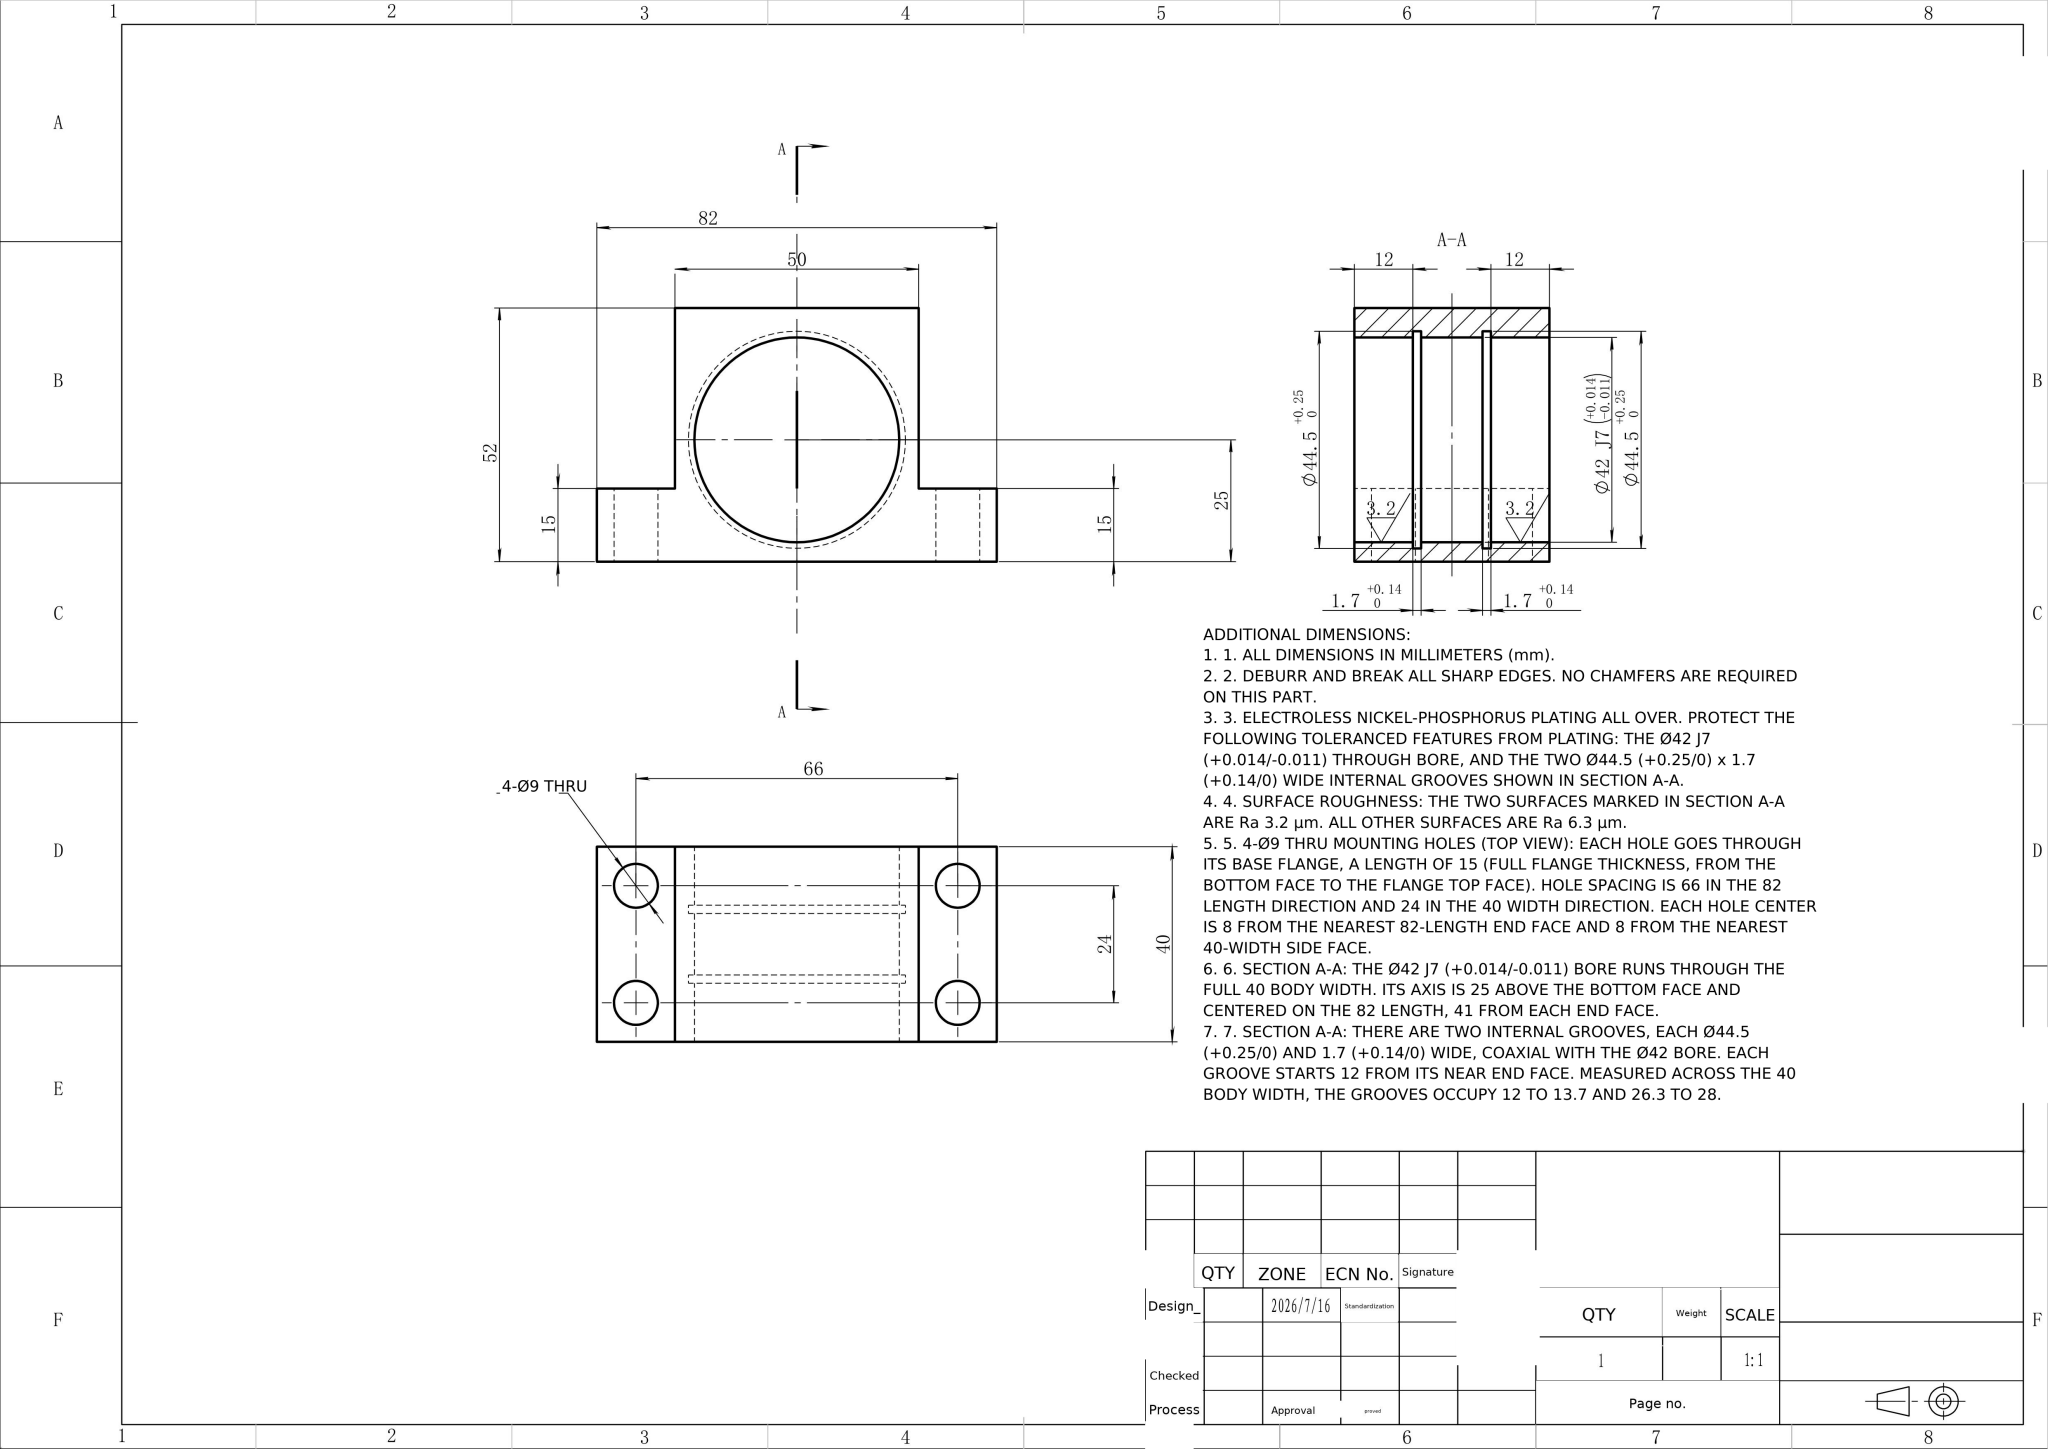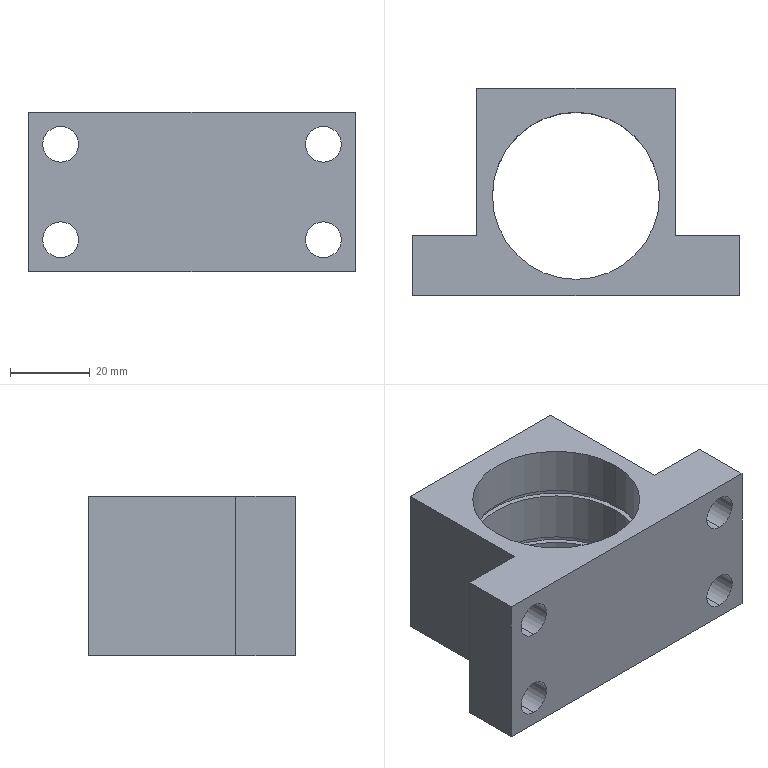Part | NX | mm | 1 solid | 32 faces | box 82 x 52 x 40 mm | volume 63388 mm3 | cylinder 18 | plane 14 | commonest cylinder face diameters 9 x8 42 x6 44.5 x4
STEP:
#1=COLOUR_RGB('',1.,1.,1.);
#2=FILL_AREA_STYLE_COLOUR('',#1);
#3=FILL_AREA_STYLE('',(#2));
#4=SURFACE_STYLE_FILL_AREA(#3);
#5=SURFACE_SIDE_STYLE('',(#4));
#6=SURFACE_STYLE_USAGE(.BOTH.,#5);
#7=PRESENTATION_STYLE_ASSIGNMENT((#6));
#8=CARTESIAN_POINT('',(74.,0.,27.5));
#9=VERTEX_POINT('',#8);
#10=CARTESIAN_POINT('',(74.,0.,36.5));
#11=VERTEX_POINT('',#10);
#12=CARTESIAN_POINT('',(74.,0.,32.));
#13=DIRECTION('',(0.,1.,0.));
#14=DIRECTION('',(0.,0.,-1.));
#15=AXIS2_PLACEMENT_3D('',#12,#13,#14);
#16=CIRCLE('',#15,4.5);
#17=EDGE_CURVE('',#9,#11,#16,.T.);
#18=ORIENTED_EDGE('',*,*,#17,.F.);
#19=CARTESIAN_POINT('',(74.,15.,27.5));
#20=VERTEX_POINT('',#19);
#21=CARTESIAN_POINT('',(74.,-0.001,27.5));
#22=DIRECTION('',(0.,1.,0.));
#23=VECTOR('',#22,1000.);
#24=LINE('',#21,#23);
#25=EDGE_CURVE('',#9,#20,#24,.T.);
#26=ORIENTED_EDGE('',*,*,#25,.T.);
#27=CARTESIAN_POINT('',(74.,15.,36.5));
#28=VERTEX_POINT('',#27);
#29=CARTESIAN_POINT('',(74.,15.,32.));
#30=DIRECTION('',(0.,1.,0.));
#31=DIRECTION('',(0.,0.,1.));
#32=AXIS2_PLACEMENT_3D('',#29,#30,#31);
#33=CIRCLE('',#32,4.5);
#34=EDGE_CURVE('',#20,#28,#33,.T.);
#35=ORIENTED_EDGE('',*,*,#34,.T.);
#36=CARTESIAN_POINT('',(74.,-0.001,36.5));
#37=DIRECTION('',(0.,1.,0.));
#38=VECTOR('',#37,1000.);
#39=LINE('',#36,#38);
#40=EDGE_CURVE('',#11,#28,#39,.T.);
#41=ORIENTED_EDGE('',*,*,#40,.F.);
#42=EDGE_LOOP('',(#18,#26,#35,#41));
#43=FACE_OUTER_BOUND('',#42,.T.);
#44=CARTESIAN_POINT('',(74.,-0.001,32.));
#45=DIRECTION('',(0.,1.,0.));
#46=DIRECTION('',(0.,0.,1.));
#47=AXIS2_PLACEMENT_3D('',#44,#45,#46);
#48=CYLINDRICAL_SURFACE('',#47,4.5);
#49=ADVANCED_FACE('',(#43),#48,.F.);
#50=CARTESIAN_POINT('',(74.,0.,3.5));
#51=VERTEX_POINT('',#50);
#52=CARTESIAN_POINT('',(74.,0.,12.5));
#53=VERTEX_POINT('',#52);
#54=CARTESIAN_POINT('',(74.,0.,8.));
#55=DIRECTION('',(0.,1.,0.));
#56=DIRECTION('',(0.,0.,-1.));
#57=AXIS2_PLACEMENT_3D('',#54,#55,#56);
#58=CIRCLE('',#57,4.5);
#59=EDGE_CURVE('',#51,#53,#58,.T.);
#60=ORIENTED_EDGE('',*,*,#59,.F.);
#61=CARTESIAN_POINT('',(74.,15.,3.5));
#62=VERTEX_POINT('',#61);
#63=CARTESIAN_POINT('',(74.,-0.001,3.5));
#64=DIRECTION('',(0.,1.,0.));
#65=VECTOR('',#64,1000.);
#66=LINE('',#63,#65);
#67=EDGE_CURVE('',#51,#62,#66,.T.);
#68=ORIENTED_EDGE('',*,*,#67,.T.);
#69=CARTESIAN_POINT('',(74.,15.,12.5));
#70=VERTEX_POINT('',#69);
#71=CARTESIAN_POINT('',(74.,15.,8.));
#72=DIRECTION('',(0.,1.,0.));
#73=DIRECTION('',(0.,0.,1.));
#74=AXIS2_PLACEMENT_3D('',#71,#72,#73);
#75=CIRCLE('',#74,4.5);
#76=EDGE_CURVE('',#62,#70,#75,.T.);
#77=ORIENTED_EDGE('',*,*,#76,.T.);
#78=CARTESIAN_POINT('',(74.,-0.001,12.5));
#79=DIRECTION('',(0.,1.,0.));
#80=VECTOR('',#79,1000.);
#81=LINE('',#78,#80);
#82=EDGE_CURVE('',#53,#70,#81,.T.);
#83=ORIENTED_EDGE('',*,*,#82,.F.);
#84=EDGE_LOOP('',(#60,#68,#77,#83));
#85=FACE_OUTER_BOUND('',#84,.T.);
#86=CARTESIAN_POINT('',(74.,-0.001,8.));
#87=DIRECTION('',(0.,1.,0.));
#88=DIRECTION('',(0.,0.,1.));
#89=AXIS2_PLACEMENT_3D('',#86,#87,#88);
#90=CYLINDRICAL_SURFACE('',#89,4.5);
#91=ADVANCED_FACE('',(#85),#90,.F.);
#92=CARTESIAN_POINT('',(8.,0.,27.5));
#93=VERTEX_POINT('',#92);
#94=CARTESIAN_POINT('',(8.,0.,36.5));
#95=VERTEX_POINT('',#94);
#96=CARTESIAN_POINT('',(8.,0.,32.));
#97=DIRECTION('',(0.,1.,0.));
#98=DIRECTION('',(0.,0.,-1.));
#99=AXIS2_PLACEMENT_3D('',#96,#97,#98);
#100=CIRCLE('',#99,4.5);
#101=EDGE_CURVE('',#93,#95,#100,.T.);
#102=ORIENTED_EDGE('',*,*,#101,.F.);
#103=CARTESIAN_POINT('',(8.,15.,27.5));
#104=VERTEX_POINT('',#103);
#105=CARTESIAN_POINT('',(8.,-0.001,27.5));
#106=DIRECTION('',(0.,1.,0.));
#107=VECTOR('',#106,1000.);
#108=LINE('',#105,#107);
#109=EDGE_CURVE('',#93,#104,#108,.T.);
#110=ORIENTED_EDGE('',*,*,#109,.T.);
#111=CARTESIAN_POINT('',(8.,15.,36.5));
#112=VERTEX_POINT('',#111);
#113=CARTESIAN_POINT('',(8.,15.,32.));
#114=DIRECTION('',(0.,1.,0.));
#115=DIRECTION('',(0.,0.,1.));
#116=AXIS2_PLACEMENT_3D('',#113,#114,#115);
#117=CIRCLE('',#116,4.5);
#118=EDGE_CURVE('',#104,#112,#117,.T.);
#119=ORIENTED_EDGE('',*,*,#118,.T.);
#120=CARTESIAN_POINT('',(8.,-0.001,36.5));
#121=DIRECTION('',(0.,1.,0.));
#122=VECTOR('',#121,1000.);
#123=LINE('',#120,#122);
#124=EDGE_CURVE('',#95,#112,#123,.T.);
#125=ORIENTED_EDGE('',*,*,#124,.F.);
#126=EDGE_LOOP('',(#102,#110,#119,#125));
#127=FACE_OUTER_BOUND('',#126,.T.);
#128=CARTESIAN_POINT('',(8.,-0.001,32.));
#129=DIRECTION('',(0.,1.,0.));
#130=DIRECTION('',(0.,0.,1.));
#131=AXIS2_PLACEMENT_3D('',#128,#129,#130);
#132=CYLINDRICAL_SURFACE('',#131,4.5);
#133=ADVANCED_FACE('',(#127),#132,.F.);
#134=CARTESIAN_POINT('',(8.,0.,3.5));
#135=VERTEX_POINT('',#134);
#136=CARTESIAN_POINT('',(8.,0.,12.5));
#137=VERTEX_POINT('',#136);
#138=CARTESIAN_POINT('',(8.,0.,8.));
#139=DIRECTION('',(0.,1.,0.));
#140=DIRECTION('',(0.,0.,-1.));
#141=AXIS2_PLACEMENT_3D('',#138,#139,#140);
#142=CIRCLE('',#141,4.5);
#143=EDGE_CURVE('',#135,#137,#142,.T.);
#144=ORIENTED_EDGE('',*,*,#143,.F.);
#145=CARTESIAN_POINT('',(8.,15.,3.5));
#146=VERTEX_POINT('',#145);
#147=CARTESIAN_POINT('',(8.,-0.001,3.5));
#148=DIRECTION('',(0.,1.,0.));
#149=VECTOR('',#148,1000.);
#150=LINE('',#147,#149);
#151=EDGE_CURVE('',#135,#146,#150,.T.);
#152=ORIENTED_EDGE('',*,*,#151,.T.);
#153=CARTESIAN_POINT('',(8.,15.,12.5));
#154=VERTEX_POINT('',#153);
#155=CARTESIAN_POINT('',(8.,15.,8.));
#156=DIRECTION('',(0.,1.,0.));
#157=DIRECTION('',(0.,0.,1.));
#158=AXIS2_PLACEMENT_3D('',#155,#156,#157);
#159=CIRCLE('',#158,4.5);
#160=EDGE_CURVE('',#146,#154,#159,.T.);
#161=ORIENTED_EDGE('',*,*,#160,.T.);
#162=CARTESIAN_POINT('',(8.,-0.001,12.5));
#163=DIRECTION('',(0.,1.,0.));
#164=VECTOR('',#163,1000.);
#165=LINE('',#162,#164);
#166=EDGE_CURVE('',#137,#154,#165,.T.);
#167=ORIENTED_EDGE('',*,*,#166,.F.);
#168=EDGE_LOOP('',(#144,#152,#161,#167));
#169=FACE_OUTER_BOUND('',#168,.T.);
#170=CARTESIAN_POINT('',(8.,-0.001,8.));
#171=DIRECTION('',(0.,1.,0.));
#172=DIRECTION('',(0.,0.,1.));
#173=AXIS2_PLACEMENT_3D('',#170,#171,#172);
#174=CYLINDRICAL_SURFACE('',#173,4.5);
#175=ADVANCED_FACE('',(#169),#174,.F.);
#176=CARTESIAN_POINT('',(20.,25.,0.));
#177=VERTEX_POINT('',#176);
#178=CARTESIAN_POINT('',(62.,25.,0.));
#179=VERTEX_POINT('',#178);
#180=CARTESIAN_POINT('',(41.,25.,0.));
#181=DIRECTION('',(0.,0.,1.));
#182=DIRECTION('',(1.,0.,0.));
#183=AXIS2_PLACEMENT_3D('',#180,#181,#182);
#184=CIRCLE('',#183,21.);
#185=EDGE_CURVE('',#177,#179,#184,.T.);
#186=ORIENTED_EDGE('',*,*,#185,.F.);
#187=CARTESIAN_POINT('',(20.,25.,12.));
#188=VERTEX_POINT('',#187);
#189=CARTESIAN_POINT('',(20.,25.,0.));
#190=DIRECTION('',(0.,0.,1.));
#191=VECTOR('',#190,1000.);
#192=LINE('',#189,#191);
#193=EDGE_CURVE('',#177,#188,#192,.T.);
#194=ORIENTED_EDGE('',*,*,#193,.T.);
#195=CARTESIAN_POINT('',(62.,25.,12.));
#196=VERTEX_POINT('',#195);
#197=CARTESIAN_POINT('',(41.,25.,12.));
#198=DIRECTION('',(0.,0.,1.));
#199=DIRECTION('',(1.,0.,0.));
#200=AXIS2_PLACEMENT_3D('',#197,#198,#199);
#201=CIRCLE('',#200,21.);
#202=EDGE_CURVE('',#188,#196,#201,.T.);
#203=ORIENTED_EDGE('',*,*,#202,.T.);
#204=CARTESIAN_POINT('',(62.,25.,0.));
#205=DIRECTION('',(0.,0.,1.));
#206=VECTOR('',#205,1000.);
#207=LINE('',#204,#206);
#208=EDGE_CURVE('',#179,#196,#207,.T.);
#209=ORIENTED_EDGE('',*,*,#208,.F.);
#210=EDGE_LOOP('',(#186,#194,#203,#209));
#211=FACE_OUTER_BOUND('',#210,.T.);
#212=CARTESIAN_POINT('',(41.,25.,0.));
#213=DIRECTION('',(0.,0.,1.));
#214=DIRECTION('',(1.,0.,0.));
#215=AXIS2_PLACEMENT_3D('',#212,#213,#214);
#216=CYLINDRICAL_SURFACE('',#215,21.);
#217=ADVANCED_FACE('',(#211),#216,.F.);
#218=CARTESIAN_POINT('',(18.75,25.,12.));
#219=VERTEX_POINT('',#218);
#220=CARTESIAN_POINT('',(63.25,25.,12.));
#221=VERTEX_POINT('',#220);
#222=CARTESIAN_POINT('',(41.,25.,12.));
#223=DIRECTION('',(0.,0.,1.));
#224=DIRECTION('',(1.,0.,0.));
#225=AXIS2_PLACEMENT_3D('',#222,#223,#224);
#226=CIRCLE('',#225,22.25);
#227=EDGE_CURVE('',#219,#221,#226,.T.);
#228=ORIENTED_EDGE('',*,*,#227,.F.);
#229=CARTESIAN_POINT('',(18.75,25.,13.7));
#230=VERTEX_POINT('',#229);
#231=CARTESIAN_POINT('',(18.75,25.,12.));
#232=DIRECTION('',(0.,0.,1.));
#233=VECTOR('',#232,1000.);
#234=LINE('',#231,#233);
#235=EDGE_CURVE('',#219,#230,#234,.T.);
#236=ORIENTED_EDGE('',*,*,#235,.T.);
#237=CARTESIAN_POINT('',(63.25,25.,13.7));
#238=VERTEX_POINT('',#237);
#239=CARTESIAN_POINT('',(41.,25.,13.7));
#240=DIRECTION('',(0.,0.,1.));
#241=DIRECTION('',(1.,0.,0.));
#242=AXIS2_PLACEMENT_3D('',#239,#240,#241);
#243=CIRCLE('',#242,22.25);
#244=EDGE_CURVE('',#230,#238,#243,.T.);
#245=ORIENTED_EDGE('',*,*,#244,.T.);
#246=CARTESIAN_POINT('',(63.25,25.,12.));
#247=DIRECTION('',(0.,0.,1.));
#248=VECTOR('',#247,1000.);
#249=LINE('',#246,#248);
#250=EDGE_CURVE('',#221,#238,#249,.T.);
#251=ORIENTED_EDGE('',*,*,#250,.F.);
#252=EDGE_LOOP('',(#228,#236,#245,#251));
#253=FACE_OUTER_BOUND('',#252,.T.);
#254=CARTESIAN_POINT('',(41.,25.,12.));
#255=DIRECTION('',(0.,0.,1.));
#256=DIRECTION('',(1.,0.,0.));
#257=AXIS2_PLACEMENT_3D('',#254,#255,#256);
#258=CYLINDRICAL_SURFACE('',#257,22.25);
#259=ADVANCED_FACE('',(#253),#258,.F.);
#260=CARTESIAN_POINT('',(62.,25.,13.7));
#261=VERTEX_POINT('',#260);
#262=CARTESIAN_POINT('',(20.,25.,13.7));
#263=VERTEX_POINT('',#262);
#264=CARTESIAN_POINT('',(41.,25.,13.7));
#265=DIRECTION('',(0.,0.,-1.));
#266=DIRECTION('',(1.,0.,0.));
#267=AXIS2_PLACEMENT_3D('',#264,#265,#266);
#268=CIRCLE('',#267,21.);
#269=EDGE_CURVE('',#261,#263,#268,.T.);
#270=ORIENTED_EDGE('',*,*,#269,.T.);
#271=CARTESIAN_POINT('',(20.,25.,26.3));
#272=VERTEX_POINT('',#271);
#273=CARTESIAN_POINT('',(20.,25.,13.7));
#274=DIRECTION('',(0.,0.,1.));
#275=VECTOR('',#274,1000.);
#276=LINE('',#273,#275);
#277=EDGE_CURVE('',#263,#272,#276,.T.);
#278=ORIENTED_EDGE('',*,*,#277,.T.);
#279=CARTESIAN_POINT('',(62.,25.,26.3));
#280=VERTEX_POINT('',#279);
#281=CARTESIAN_POINT('',(41.,25.,26.3));
#282=DIRECTION('',(0.,0.,1.));
#283=DIRECTION('',(1.,0.,0.));
#284=AXIS2_PLACEMENT_3D('',#281,#282,#283);
#285=CIRCLE('',#284,21.);
#286=EDGE_CURVE('',#272,#280,#285,.T.);
#287=ORIENTED_EDGE('',*,*,#286,.T.);
#288=CARTESIAN_POINT('',(62.,25.,13.7));
#289=DIRECTION('',(0.,0.,1.));
#290=VECTOR('',#289,1000.);
#291=LINE('',#288,#290);
#292=EDGE_CURVE('',#261,#280,#291,.T.);
#293=ORIENTED_EDGE('',*,*,#292,.F.);
#294=EDGE_LOOP('',(#270,#278,#287,#293));
#295=FACE_OUTER_BOUND('',#294,.T.);
#296=CARTESIAN_POINT('',(41.,25.,13.7));
#297=DIRECTION('',(0.,0.,1.));
#298=DIRECTION('',(1.,0.,0.));
#299=AXIS2_PLACEMENT_3D('',#296,#297,#298);
#300=CYLINDRICAL_SURFACE('',#299,21.);
#301=ADVANCED_FACE('',(#295),#300,.F.);
#302=CARTESIAN_POINT('',(18.75,25.,26.3));
#303=VERTEX_POINT('',#302);
#304=CARTESIAN_POINT('',(63.25,25.,26.3));
#305=VERTEX_POINT('',#304);
#306=CARTESIAN_POINT('',(41.,25.,26.3));
#307=DIRECTION('',(0.,0.,1.));
#308=DIRECTION('',(1.,0.,0.));
#309=AXIS2_PLACEMENT_3D('',#306,#307,#308);
#310=CIRCLE('',#309,22.25);
#311=EDGE_CURVE('',#303,#305,#310,.T.);
#312=ORIENTED_EDGE('',*,*,#311,.F.);
#313=CARTESIAN_POINT('',(18.75,25.,28.));
#314=VERTEX_POINT('',#313);
#315=CARTESIAN_POINT('',(18.75,25.,26.3));
#316=DIRECTION('',(0.,0.,1.));
#317=VECTOR('',#316,1000.);
#318=LINE('',#315,#317);
#319=EDGE_CURVE('',#303,#314,#318,.T.);
#320=ORIENTED_EDGE('',*,*,#319,.T.);
#321=CARTESIAN_POINT('',(63.25,25.,28.));
#322=VERTEX_POINT('',#321);
#323=CARTESIAN_POINT('',(41.,25.,28.));
#324=DIRECTION('',(0.,0.,1.));
#325=DIRECTION('',(1.,0.,0.));
#326=AXIS2_PLACEMENT_3D('',#323,#324,#325);
#327=CIRCLE('',#326,22.25);
#328=EDGE_CURVE('',#314,#322,#327,.T.);
#329=ORIENTED_EDGE('',*,*,#328,.T.);
#330=CARTESIAN_POINT('',(63.25,25.,26.3));
#331=DIRECTION('',(0.,0.,1.));
#332=VECTOR('',#331,1000.);
#333=LINE('',#330,#332);
#334=EDGE_CURVE('',#305,#322,#333,.T.);
#335=ORIENTED_EDGE('',*,*,#334,.F.);
#336=EDGE_LOOP('',(#312,#320,#329,#335));
#337=FACE_OUTER_BOUND('',#336,.T.);
#338=CARTESIAN_POINT('',(41.,25.,26.3));
#339=DIRECTION('',(0.,0.,1.));
#340=DIRECTION('',(1.,0.,0.));
#341=AXIS2_PLACEMENT_3D('',#338,#339,#340);
#342=CYLINDRICAL_SURFACE('',#341,22.25);
#343=ADVANCED_FACE('',(#337),#342,.F.);
#344=CARTESIAN_POINT('',(62.,25.,28.));
#345=VERTEX_POINT('',#344);
#346=CARTESIAN_POINT('',(20.,25.,28.));
#347=VERTEX_POINT('',#346);
#348=CARTESIAN_POINT('',(41.,25.,28.));
#349=DIRECTION('',(0.,0.,-1.));
#350=DIRECTION('',(1.,0.,0.));
#351=AXIS2_PLACEMENT_3D('',#348,#349,#350);
#352=CIRCLE('',#351,21.);
#353=EDGE_CURVE('',#345,#347,#352,.T.);
#354=ORIENTED_EDGE('',*,*,#353,.T.);
#355=CARTESIAN_POINT('',(20.,25.,40.));
#356=VERTEX_POINT('',#355);
#357=CARTESIAN_POINT('',(20.,25.,28.));
#358=DIRECTION('',(0.,0.,1.));
#359=VECTOR('',#358,1000.);
#360=LINE('',#357,#359);
#361=EDGE_CURVE('',#347,#356,#360,.T.);
#362=ORIENTED_EDGE('',*,*,#361,.T.);
#363=CARTESIAN_POINT('',(62.,25.,40.));
#364=VERTEX_POINT('',#363);
#365=CARTESIAN_POINT('',(41.,25.,40.));
#366=DIRECTION('',(0.,0.,1.));
#367=DIRECTION('',(1.,0.,0.));
#368=AXIS2_PLACEMENT_3D('',#365,#366,#367);
#369=CIRCLE('',#368,21.);
#370=EDGE_CURVE('',#356,#364,#369,.T.);
#371=ORIENTED_EDGE('',*,*,#370,.T.);
#372=CARTESIAN_POINT('',(62.,25.,28.));
#373=DIRECTION('',(0.,0.,1.));
#374=VECTOR('',#373,1000.);
#375=LINE('',#372,#374);
#376=EDGE_CURVE('',#345,#364,#375,.T.);
#377=ORIENTED_EDGE('',*,*,#376,.F.);
#378=EDGE_LOOP('',(#354,#362,#371,#377));
#379=FACE_OUTER_BOUND('',#378,.T.);
#380=CARTESIAN_POINT('',(41.,25.,28.));
#381=DIRECTION('',(0.,0.,1.));
#382=DIRECTION('',(1.,0.,0.));
#383=AXIS2_PLACEMENT_3D('',#380,#381,#382);
#384=CYLINDRICAL_SURFACE('',#383,21.);
#385=ADVANCED_FACE('',(#379),#384,.F.);
#386=CARTESIAN_POINT('',(16.,15.,0.));
#387=VERTEX_POINT('',#386);
#388=CARTESIAN_POINT('',(16.,52.,0.));
#389=VERTEX_POINT('',#388);
#390=CARTESIAN_POINT('',(16.,30.857,0.));
#391=DIRECTION('',(-0.,1.,0.));
#392=VECTOR('',#391,1000.);
#393=LINE('',#390,#392);
#394=EDGE_CURVE('',#387,#389,#393,.T.);
#395=ORIENTED_EDGE('',*,*,#394,.F.);
#396=CARTESIAN_POINT('',(16.,15.,40.));
#397=VERTEX_POINT('',#396);
#398=CARTESIAN_POINT('',(16.,15.,40.));
#399=DIRECTION('',(0.,0.,-1.));
#400=VECTOR('',#399,1000.);
#401=LINE('',#398,#400);
#402=EDGE_CURVE('',#397,#387,#401,.T.);
#403=ORIENTED_EDGE('',*,*,#402,.F.);
#404=CARTESIAN_POINT('',(16.,52.,40.));
#405=VERTEX_POINT('',#404);
#406=CARTESIAN_POINT('',(16.,30.857,40.));
#407=DIRECTION('',(-0.,1.,0.));
#408=VECTOR('',#407,1000.);
#409=LINE('',#406,#408);
#410=EDGE_CURVE('',#397,#405,#409,.T.);
#411=ORIENTED_EDGE('',*,*,#410,.T.);
#412=CARTESIAN_POINT('',(16.,52.,40.));
#413=DIRECTION('',(0.,0.,-1.));
#414=VECTOR('',#413,1000.);
#415=LINE('',#412,#414);
#416=EDGE_CURVE('',#405,#389,#415,.T.);
#417=ORIENTED_EDGE('',*,*,#416,.T.);
#418=EDGE_LOOP('',(#395,#403,#411,#417));
#419=FACE_OUTER_BOUND('',#418,.T.);
#420=CARTESIAN_POINT('',(16.,30.857,40.));
#421=DIRECTION('',(-1.,-0.,0.));
#422=DIRECTION('',(0.,-1.,0.));
#423=AXIS2_PLACEMENT_3D('',#420,#421,#422);
#424=PLANE('',#423);
#425=ADVANCED_FACE('',(#419),#424,.T.);
#426=CARTESIAN_POINT('',(8.,15.,32.));
#427=DIRECTION('',(0.,1.,0.));
#428=DIRECTION('',(0.,0.,1.));
#429=AXIS2_PLACEMENT_3D('',#426,#427,#428);
#430=CIRCLE('',#429,4.5);
#431=EDGE_CURVE('',#112,#104,#430,.T.);
#432=ORIENTED_EDGE('',*,*,#431,.F.);
#433=ORIENTED_EDGE('',*,*,#118,.F.);
#434=EDGE_LOOP('',(#432,#433));
#435=FACE_BOUND('',#434,.T.);
#436=CARTESIAN_POINT('',(8.,15.,8.));
#437=DIRECTION('',(0.,1.,0.));
#438=DIRECTION('',(0.,0.,1.));
#439=AXIS2_PLACEMENT_3D('',#436,#437,#438);
#440=CIRCLE('',#439,4.5);
#441=EDGE_CURVE('',#154,#146,#440,.T.);
#442=ORIENTED_EDGE('',*,*,#441,.F.);
#443=ORIENTED_EDGE('',*,*,#160,.F.);
#444=EDGE_LOOP('',(#442,#443));
#445=FACE_BOUND('',#444,.T.);
#446=CARTESIAN_POINT('',(0.,15.,0.));
#447=VERTEX_POINT('',#446);
#448=CARTESIAN_POINT('',(-52.458,15.,0.));
#449=DIRECTION('',(-1.,0.,0.));
#450=VECTOR('',#449,1000.);
#451=LINE('',#448,#450);
#452=EDGE_CURVE('',#387,#447,#451,.T.);
#453=ORIENTED_EDGE('',*,*,#452,.T.);
#454=CARTESIAN_POINT('',(0.,15.,40.));
#455=VERTEX_POINT('',#454);
#456=CARTESIAN_POINT('',(0.,15.,40.));
#457=DIRECTION('',(0.,0.,-1.));
#458=VECTOR('',#457,1000.);
#459=LINE('',#456,#458);
#460=EDGE_CURVE('',#455,#447,#459,.T.);
#461=ORIENTED_EDGE('',*,*,#460,.F.);
#462=CARTESIAN_POINT('',(-52.458,15.,40.));
#463=DIRECTION('',(-1.,0.,0.));
#464=VECTOR('',#463,1000.);
#465=LINE('',#462,#464);
#466=EDGE_CURVE('',#397,#455,#465,.T.);
#467=ORIENTED_EDGE('',*,*,#466,.F.);
#468=ORIENTED_EDGE('',*,*,#402,.T.);
#469=EDGE_LOOP('',(#453,#461,#467,#468));
#470=FACE_OUTER_BOUND('',#469,.T.);
#471=CARTESIAN_POINT('',(-52.458,15.,40.));
#472=DIRECTION('',(0.,-1.,0.));
#473=DIRECTION('',(0.,0.,-1.));
#474=AXIS2_PLACEMENT_3D('',#471,#472,#473);
#475=PLANE('',#474);
#476=ADVANCED_FACE('',(#435,#445,#470),#475,.F.);
#477=CARTESIAN_POINT('',(0.,0.,0.));
#478=VERTEX_POINT('',#477);
#479=CARTESIAN_POINT('',(0.,30.857,0.));
#480=DIRECTION('',(0.,-1.,0.));
#481=VECTOR('',#480,1000.);
#482=LINE('',#479,#481);
#483=EDGE_CURVE('',#447,#478,#482,.T.);
#484=ORIENTED_EDGE('',*,*,#483,.T.);
#485=CARTESIAN_POINT('',(0.,0.,40.));
#486=VERTEX_POINT('',#485);
#487=CARTESIAN_POINT('',(0.,0.,40.));
#488=DIRECTION('',(0.,0.,-1.));
#489=VECTOR('',#488,1000.);
#490=LINE('',#487,#489);
#491=EDGE_CURVE('',#486,#478,#490,.T.);
#492=ORIENTED_EDGE('',*,*,#491,.F.);
#493=CARTESIAN_POINT('',(0.,30.857,40.));
#494=DIRECTION('',(0.,-1.,0.));
#495=VECTOR('',#494,1000.);
#496=LINE('',#493,#495);
#497=EDGE_CURVE('',#455,#486,#496,.T.);
#498=ORIENTED_EDGE('',*,*,#497,.F.);
#499=ORIENTED_EDGE('',*,*,#460,.T.);
#500=EDGE_LOOP('',(#484,#492,#498,#499));
#501=FACE_OUTER_BOUND('',#500,.T.);
#502=CARTESIAN_POINT('',(0.,30.857,40.));
#503=DIRECTION('',(1.,0.,0.));
#504=DIRECTION('',(0.,0.,-1.));
#505=AXIS2_PLACEMENT_3D('',#502,#503,#504);
#506=PLANE('',#505);
#507=ADVANCED_FACE('',(#501),#506,.F.);
#508=CARTESIAN_POINT('',(74.,0.,32.));
#509=DIRECTION('',(0.,1.,0.));
#510=DIRECTION('',(0.,0.,-1.));
#511=AXIS2_PLACEMENT_3D('',#508,#509,#510);
#512=CIRCLE('',#511,4.5);
#513=EDGE_CURVE('',#11,#9,#512,.T.);
#514=ORIENTED_EDGE('',*,*,#513,.T.);
#515=ORIENTED_EDGE('',*,*,#17,.T.);
#516=EDGE_LOOP('',(#514,#515));
#517=FACE_BOUND('',#516,.T.);
#518=CARTESIAN_POINT('',(74.,0.,8.));
#519=DIRECTION('',(0.,1.,0.));
#520=DIRECTION('',(0.,0.,-1.));
#521=AXIS2_PLACEMENT_3D('',#518,#519,#520);
#522=CIRCLE('',#521,4.5);
#523=EDGE_CURVE('',#53,#51,#522,.T.);
#524=ORIENTED_EDGE('',*,*,#523,.T.);
#525=ORIENTED_EDGE('',*,*,#59,.T.);
#526=EDGE_LOOP('',(#524,#525));
#527=FACE_BOUND('',#526,.T.);
#528=CARTESIAN_POINT('',(8.,0.,32.));
#529=DIRECTION('',(0.,1.,0.));
#530=DIRECTION('',(0.,0.,-1.));
#531=AXIS2_PLACEMENT_3D('',#528,#529,#530);
#532=CIRCLE('',#531,4.5);
#533=EDGE_CURVE('',#95,#93,#532,.T.);
#534=ORIENTED_EDGE('',*,*,#533,.T.);
#535=ORIENTED_EDGE('',*,*,#101,.T.);
#536=EDGE_LOOP('',(#534,#535));
#537=FACE_BOUND('',#536,.T.);
#538=CARTESIAN_POINT('',(8.,0.,8.));
#539=DIRECTION('',(0.,1.,0.));
#540=DIRECTION('',(0.,0.,-1.));
#541=AXIS2_PLACEMENT_3D('',#538,#539,#540);
#542=CIRCLE('',#541,4.5);
#543=EDGE_CURVE('',#137,#135,#542,.T.);
#544=ORIENTED_EDGE('',*,*,#543,.T.);
#545=ORIENTED_EDGE('',*,*,#143,.T.);
#546=EDGE_LOOP('',(#544,#545));
#547=FACE_BOUND('',#546,.T.);
#548=CARTESIAN_POINT('',(82.,0.,0.));
#549=VERTEX_POINT('',#548);
#550=CARTESIAN_POINT('',(-52.458,0.,0.));
#551=DIRECTION('',(-1.,0.,0.));
#552=VECTOR('',#551,1000.);
#553=LINE('',#550,#552);
#554=EDGE_CURVE('',#549,#478,#553,.T.);
#555=ORIENTED_EDGE('',*,*,#554,.F.);
#556=CARTESIAN_POINT('',(82.,0.,40.));
#557=VERTEX_POINT('',#556);
#558=CARTESIAN_POINT('',(82.,0.,40.));
#559=DIRECTION('',(0.,0.,-1.));
#560=VECTOR('',#559,1000.);
#561=LINE('',#558,#560);
#562=EDGE_CURVE('',#557,#549,#561,.T.);
#563=ORIENTED_EDGE('',*,*,#562,.F.);
#564=CARTESIAN_POINT('',(-52.458,0.,40.));
#565=DIRECTION('',(-1.,0.,0.));
#566=VECTOR('',#565,1000.);
#567=LINE('',#564,#566);
#568=EDGE_CURVE('',#557,#486,#567,.T.);
#569=ORIENTED_EDGE('',*,*,#568,.T.);
#570=ORIENTED_EDGE('',*,*,#491,.T.);
#571=EDGE_LOOP('',(#555,#563,#569,#570));
#572=FACE_OUTER_BOUND('',#571,.T.);
#573=CARTESIAN_POINT('',(-52.458,0.,40.));
#574=DIRECTION('',(0.,-1.,0.));
#575=DIRECTION('',(0.,0.,-1.));
#576=AXIS2_PLACEMENT_3D('',#573,#574,#575);
#577=PLANE('',#576);
#578=ADVANCED_FACE('',(#517,#527,#537,#547,#572),#577,.T.);
#579=CARTESIAN_POINT('',(82.,15.,0.));
#580=VERTEX_POINT('',#579);
#581=CARTESIAN_POINT('',(82.,30.857,0.));
#582=DIRECTION('',(0.,-1.,0.));
#583=VECTOR('',#582,1000.);
#584=LINE('',#581,#583);
#585=EDGE_CURVE('',#580,#549,#584,.T.);
#586=ORIENTED_EDGE('',*,*,#585,.F.);
#587=CARTESIAN_POINT('',(82.,15.,40.));
#588=VERTEX_POINT('',#587);
#589=CARTESIAN_POINT('',(82.,15.,40.));
#590=DIRECTION('',(0.,0.,-1.));
#591=VECTOR('',#590,1000.);
#592=LINE('',#589,#591);
#593=EDGE_CURVE('',#588,#580,#592,.T.);
#594=ORIENTED_EDGE('',*,*,#593,.F.);
#595=CARTESIAN_POINT('',(82.,30.857,40.));
#596=DIRECTION('',(0.,-1.,0.));
#597=VECTOR('',#596,1000.);
#598=LINE('',#595,#597);
#599=EDGE_CURVE('',#588,#557,#598,.T.);
#600=ORIENTED_EDGE('',*,*,#599,.T.);
#601=ORIENTED_EDGE('',*,*,#562,.T.);
#602=EDGE_LOOP('',(#586,#594,#600,#601));
#603=FACE_OUTER_BOUND('',#602,.T.);
#604=CARTESIAN_POINT('',(82.,30.857,40.));
#605=DIRECTION('',(1.,0.,0.));
#606=DIRECTION('',(0.,0.,-1.));
#607=AXIS2_PLACEMENT_3D('',#604,#605,#606);
#608=PLANE('',#607);
#609=ADVANCED_FACE('',(#603),#608,.T.);
#610=CARTESIAN_POINT('',(74.,15.,32.));
#611=DIRECTION('',(0.,1.,0.));
#612=DIRECTION('',(0.,0.,1.));
#613=AXIS2_PLACEMENT_3D('',#610,#611,#612);
#614=CIRCLE('',#613,4.5);
#615=EDGE_CURVE('',#28,#20,#614,.T.);
#616=ORIENTED_EDGE('',*,*,#615,.F.);
#617=ORIENTED_EDGE('',*,*,#34,.F.);
#618=EDGE_LOOP('',(#616,#617));
#619=FACE_BOUND('',#618,.T.);
#620=CARTESIAN_POINT('',(74.,15.,8.));
#621=DIRECTION('',(0.,1.,0.));
#622=DIRECTION('',(0.,0.,1.));
#623=AXIS2_PLACEMENT_3D('',#620,#621,#622);
#624=CIRCLE('',#623,4.5);
#625=EDGE_CURVE('',#70,#62,#624,.T.);
#626=ORIENTED_EDGE('',*,*,#625,.F.);
#627=ORIENTED_EDGE('',*,*,#76,.F.);
#628=EDGE_LOOP('',(#626,#627));
#629=FACE_BOUND('',#628,.T.);
#630=CARTESIAN_POINT('',(66.,15.,0.));
#631=VERTEX_POINT('',#630);
#632=CARTESIAN_POINT('',(-52.458,15.,0.));
#633=DIRECTION('',(-1.,0.,0.));
#634=VECTOR('',#633,1000.);
#635=LINE('',#632,#634);
#636=EDGE_CURVE('',#580,#631,#635,.T.);
#637=ORIENTED_EDGE('',*,*,#636,.T.);
#638=CARTESIAN_POINT('',(66.,15.,40.));
#639=VERTEX_POINT('',#638);
#640=CARTESIAN_POINT('',(66.,15.,40.));
#641=DIRECTION('',(0.,0.,-1.));
#642=VECTOR('',#641,1000.);
#643=LINE('',#640,#642);
#644=EDGE_CURVE('',#639,#631,#643,.T.);
#645=ORIENTED_EDGE('',*,*,#644,.F.);
#646=CARTESIAN_POINT('',(-52.458,15.,40.));
#647=DIRECTION('',(-1.,0.,0.));
#648=VECTOR('',#647,1000.);
#649=LINE('',#646,#648);
#650=EDGE_CURVE('',#588,#639,#649,.T.);
#651=ORIENTED_EDGE('',*,*,#650,.F.);
#652=ORIENTED_EDGE('',*,*,#593,.T.);
#653=EDGE_LOOP('',(#637,#645,#651,#652));
#654=FACE_OUTER_BOUND('',#653,.T.);
#655=CARTESIAN_POINT('',(-52.458,15.,40.));
#656=DIRECTION('',(0.,-1.,0.));
#657=DIRECTION('',(0.,0.,-1.));
#658=AXIS2_PLACEMENT_3D('',#655,#656,#657);
#659=PLANE('',#658);
#660=ADVANCED_FACE('',(#619,#629,#654),#659,.F.);
#661=CARTESIAN_POINT('',(66.,52.,0.));
#662=VERTEX_POINT('',#661);
#663=CARTESIAN_POINT('',(66.,30.857,0.));
#664=DIRECTION('',(0.,1.,0.));
#665=VECTOR('',#664,1000.);
#666=LINE('',#663,#665);
#667=EDGE_CURVE('',#631,#662,#666,.T.);
#668=ORIENTED_EDGE('',*,*,#667,.T.);
#669=CARTESIAN_POINT('',(66.,52.,40.));
#670=VERTEX_POINT('',#669);
#671=CARTESIAN_POINT('',(66.,52.,40.));
#672=DIRECTION('',(0.,0.,-1.));
#673=VECTOR('',#672,1000.);
#674=LINE('',#671,#673);
#675=EDGE_CURVE('',#670,#662,#674,.T.);
#676=ORIENTED_EDGE('',*,*,#675,.F.);
#677=CARTESIAN_POINT('',(66.,30.857,40.));
#678=DIRECTION('',(0.,1.,0.));
#679=VECTOR('',#678,1000.);
#680=LINE('',#677,#679);
#681=EDGE_CURVE('',#639,#670,#680,.T.);
#682=ORIENTED_EDGE('',*,*,#681,.F.);
#683=ORIENTED_EDGE('',*,*,#644,.T.);
#684=EDGE_LOOP('',(#668,#676,#682,#683));
#685=FACE_OUTER_BOUND('',#684,.T.);
#686=CARTESIAN_POINT('',(66.,30.857,40.));
#687=DIRECTION('',(-1.,0.,0.));
#688=DIRECTION('',(0.,0.,1.));
#689=AXIS2_PLACEMENT_3D('',#686,#687,#688);
#690=PLANE('',#689);
#691=ADVANCED_FACE('',(#685),#690,.F.);
#692=CARTESIAN_POINT('',(-52.458,52.,0.));
#693=DIRECTION('',(-1.,0.,0.));
#694=VECTOR('',#693,1000.);
#695=LINE('',#692,#694);
#696=EDGE_CURVE('',#662,#389,#695,.T.);
#697=ORIENTED_EDGE('',*,*,#696,.T.);
#698=ORIENTED_EDGE('',*,*,#416,.F.);
#699=CARTESIAN_POINT('',(-52.458,52.,40.));
#700=DIRECTION('',(-1.,0.,0.));
#701=VECTOR('',#700,1000.);
#702=LINE('',#699,#701);
#703=EDGE_CURVE('',#670,#405,#702,.T.);
#704=ORIENTED_EDGE('',*,*,#703,.F.);
#705=ORIENTED_EDGE('',*,*,#675,.T.);
#706=EDGE_LOOP('',(#697,#698,#704,#705));
#707=FACE_OUTER_BOUND('',#706,.T.);
#708=CARTESIAN_POINT('',(-52.458,52.,40.));
#709=DIRECTION('',(0.,-1.,0.));
#710=DIRECTION('',(0.,0.,-1.));
#711=AXIS2_PLACEMENT_3D('',#708,#709,#710);
#712=PLANE('',#711);
#713=ADVANCED_FACE('',(#707),#712,.F.);
#714=CARTESIAN_POINT('',(41.,25.,40.));
#715=DIRECTION('',(0.,0.,1.));
#716=DIRECTION('',(1.,0.,0.));
#717=AXIS2_PLACEMENT_3D('',#714,#715,#716);
#718=CIRCLE('',#717,21.);
#719=EDGE_CURVE('',#364,#356,#718,.T.);
#720=ORIENTED_EDGE('',*,*,#719,.F.);
#721=ORIENTED_EDGE('',*,*,#370,.F.);
#722=EDGE_LOOP('',(#720,#721));
#723=FACE_BOUND('',#722,.T.);
#724=ORIENTED_EDGE('',*,*,#410,.F.);
#725=ORIENTED_EDGE('',*,*,#466,.T.);
#726=ORIENTED_EDGE('',*,*,#497,.T.);
#727=ORIENTED_EDGE('',*,*,#568,.F.);
#728=ORIENTED_EDGE('',*,*,#599,.F.);
#729=ORIENTED_EDGE('',*,*,#650,.T.);
#730=ORIENTED_EDGE('',*,*,#681,.T.);
#731=ORIENTED_EDGE('',*,*,#703,.T.);
#732=EDGE_LOOP('',(#724,#725,#726,#727,#728,#729,#730,#731));
#733=FACE_OUTER_BOUND('',#732,.T.);
#734=CARTESIAN_POINT('',(-52.458,30.857,40.));
#735=DIRECTION('',(0.,0.,-1.));
#736=DIRECTION('',(-1.,0.,0.));
#737=AXIS2_PLACEMENT_3D('',#734,#735,#736);
#738=PLANE('',#737);
#739=ADVANCED_FACE('',(#723,#733),#738,.F.);
#740=CARTESIAN_POINT('',(41.,25.,0.));
#741=DIRECTION('',(0.,0.,1.));
#742=DIRECTION('',(1.,0.,0.));
#743=AXIS2_PLACEMENT_3D('',#740,#741,#742);
#744=CIRCLE('',#743,21.);
#745=EDGE_CURVE('',#179,#177,#744,.T.);
#746=ORIENTED_EDGE('',*,*,#745,.T.);
#747=ORIENTED_EDGE('',*,*,#185,.T.);
#748=EDGE_LOOP('',(#746,#747));
#749=FACE_BOUND('',#748,.T.);
#750=ORIENTED_EDGE('',*,*,#394,.T.);
#751=ORIENTED_EDGE('',*,*,#696,.F.);
#752=ORIENTED_EDGE('',*,*,#667,.F.);
#753=ORIENTED_EDGE('',*,*,#636,.F.);
#754=ORIENTED_EDGE('',*,*,#585,.T.);
#755=ORIENTED_EDGE('',*,*,#554,.T.);
#756=ORIENTED_EDGE('',*,*,#483,.F.);
#757=ORIENTED_EDGE('',*,*,#452,.F.);
#758=EDGE_LOOP('',(#750,#751,#752,#753,#754,#755,#756,#757));
#759=FACE_OUTER_BOUND('',#758,.T.);
#760=CARTESIAN_POINT('',(-52.458,30.857,0.));
#761=DIRECTION('',(0.,0.,-1.));
#762=DIRECTION('',(-1.,0.,0.));
#763=AXIS2_PLACEMENT_3D('',#760,#761,#762);
#764=PLANE('',#763);
#765=ADVANCED_FACE('',(#749,#759),#764,.T.);
#766=ORIENTED_EDGE('',*,*,#361,.F.);
#767=CARTESIAN_POINT('',(41.,25.,28.));
#768=DIRECTION('',(0.,0.,-1.));
#769=DIRECTION('',(1.,0.,0.));
#770=AXIS2_PLACEMENT_3D('',#767,#768,#769);
#771=CIRCLE('',#770,21.);
#772=EDGE_CURVE('',#347,#345,#771,.T.);
#773=ORIENTED_EDGE('',*,*,#772,.T.);
#774=ORIENTED_EDGE('',*,*,#376,.T.);
#775=ORIENTED_EDGE('',*,*,#719,.T.);
#776=EDGE_LOOP('',(#766,#773,#774,#775));
#777=FACE_OUTER_BOUND('',#776,.T.);
#778=CARTESIAN_POINT('',(41.,25.,28.));
#779=DIRECTION('',(0.,0.,1.));
#780=DIRECTION('',(1.,0.,0.));
#781=AXIS2_PLACEMENT_3D('',#778,#779,#780);
#782=CYLINDRICAL_SURFACE('',#781,21.);
#783=ADVANCED_FACE('',(#777),#782,.F.);
#784=CARTESIAN_POINT('',(41.,25.,28.));
#785=DIRECTION('',(0.,0.,1.));
#786=DIRECTION('',(1.,0.,0.));
#787=AXIS2_PLACEMENT_3D('',#784,#785,#786);
#788=CIRCLE('',#787,22.25);
#789=EDGE_CURVE('',#322,#314,#788,.T.);
#790=ORIENTED_EDGE('',*,*,#789,.F.);
#791=ORIENTED_EDGE('',*,*,#328,.F.);
#792=EDGE_LOOP('',(#790,#791));
#793=FACE_OUTER_BOUND('',#792,.T.);
#794=ORIENTED_EDGE('',*,*,#353,.F.);
#795=ORIENTED_EDGE('',*,*,#772,.F.);
#796=EDGE_LOOP('',(#794,#795));
#797=FACE_BOUND('',#796,.T.);
#798=CARTESIAN_POINT('',(41.,25.,28.));
#799=DIRECTION('',(0.,0.,1.));
#800=DIRECTION('',(1.,0.,0.));
#801=AXIS2_PLACEMENT_3D('',#798,#799,#800);
#802=PLANE('',#801);
#803=ADVANCED_FACE('',(#793,#797),#802,.F.);
#804=ORIENTED_EDGE('',*,*,#319,.F.);
#805=CARTESIAN_POINT('',(41.,25.,26.3));
#806=DIRECTION('',(0.,0.,1.));
#807=DIRECTION('',(1.,0.,0.));
#808=AXIS2_PLACEMENT_3D('',#805,#806,#807);
#809=CIRCLE('',#808,22.25);
#810=EDGE_CURVE('',#305,#303,#809,.T.);
#811=ORIENTED_EDGE('',*,*,#810,.F.);
#812=ORIENTED_EDGE('',*,*,#334,.T.);
#813=ORIENTED_EDGE('',*,*,#789,.T.);
#814=EDGE_LOOP('',(#804,#811,#812,#813));
#815=FACE_OUTER_BOUND('',#814,.T.);
#816=CARTESIAN_POINT('',(41.,25.,26.3));
#817=DIRECTION('',(0.,0.,1.));
#818=DIRECTION('',(1.,0.,0.));
#819=AXIS2_PLACEMENT_3D('',#816,#817,#818);
#820=CYLINDRICAL_SURFACE('',#819,22.25);
#821=ADVANCED_FACE('',(#815),#820,.F.);
#822=CARTESIAN_POINT('',(41.,25.,26.3));
#823=DIRECTION('',(0.,0.,1.));
#824=DIRECTION('',(1.,0.,0.));
#825=AXIS2_PLACEMENT_3D('',#822,#823,#824);
#826=CIRCLE('',#825,21.);
#827=EDGE_CURVE('',#280,#272,#826,.T.);
#828=ORIENTED_EDGE('',*,*,#827,.F.);
#829=ORIENTED_EDGE('',*,*,#286,.F.);
#830=EDGE_LOOP('',(#828,#829));
#831=FACE_BOUND('',#830,.T.);
#832=ORIENTED_EDGE('',*,*,#810,.T.);
#833=ORIENTED_EDGE('',*,*,#311,.T.);
#834=EDGE_LOOP('',(#832,#833));
#835=FACE_OUTER_BOUND('',#834,.T.);
#836=CARTESIAN_POINT('',(41.,25.,26.3));
#837=DIRECTION('',(0.,0.,1.));
#838=DIRECTION('',(1.,0.,0.));
#839=AXIS2_PLACEMENT_3D('',#836,#837,#838);
#840=PLANE('',#839);
#841=ADVANCED_FACE('',(#831,#835),#840,.T.);
#842=ORIENTED_EDGE('',*,*,#277,.F.);
#843=CARTESIAN_POINT('',(41.,25.,13.7));
#844=DIRECTION('',(0.,0.,-1.));
#845=DIRECTION('',(1.,0.,0.));
#846=AXIS2_PLACEMENT_3D('',#843,#844,#845);
#847=CIRCLE('',#846,21.);
#848=EDGE_CURVE('',#263,#261,#847,.T.);
#849=ORIENTED_EDGE('',*,*,#848,.T.);
#850=ORIENTED_EDGE('',*,*,#292,.T.);
#851=ORIENTED_EDGE('',*,*,#827,.T.);
#852=EDGE_LOOP('',(#842,#849,#850,#851));
#853=FACE_OUTER_BOUND('',#852,.T.);
#854=CARTESIAN_POINT('',(41.,25.,13.7));
#855=DIRECTION('',(0.,0.,1.));
#856=DIRECTION('',(1.,0.,0.));
#857=AXIS2_PLACEMENT_3D('',#854,#855,#856);
#858=CYLINDRICAL_SURFACE('',#857,21.);
#859=ADVANCED_FACE('',(#853),#858,.F.);
#860=CARTESIAN_POINT('',(41.,25.,13.7));
#861=DIRECTION('',(0.,0.,1.));
#862=DIRECTION('',(1.,0.,0.));
#863=AXIS2_PLACEMENT_3D('',#860,#861,#862);
#864=CIRCLE('',#863,22.25);
#865=EDGE_CURVE('',#238,#230,#864,.T.);
#866=ORIENTED_EDGE('',*,*,#865,.F.);
#867=ORIENTED_EDGE('',*,*,#244,.F.);
#868=EDGE_LOOP('',(#866,#867));
#869=FACE_OUTER_BOUND('',#868,.T.);
#870=ORIENTED_EDGE('',*,*,#269,.F.);
#871=ORIENTED_EDGE('',*,*,#848,.F.);
#872=EDGE_LOOP('',(#870,#871));
#873=FACE_BOUND('',#872,.T.);
#874=CARTESIAN_POINT('',(41.,25.,13.7));
#875=DIRECTION('',(0.,0.,1.));
#876=DIRECTION('',(1.,0.,0.));
#877=AXIS2_PLACEMENT_3D('',#874,#875,#876);
#878=PLANE('',#877);
#879=ADVANCED_FACE('',(#869,#873),#878,.F.);
#880=ORIENTED_EDGE('',*,*,#235,.F.);
#881=CARTESIAN_POINT('',(41.,25.,12.));
#882=DIRECTION('',(0.,0.,1.));
#883=DIRECTION('',(1.,0.,0.));
#884=AXIS2_PLACEMENT_3D('',#881,#882,#883);
#885=CIRCLE('',#884,22.25);
#886=EDGE_CURVE('',#221,#219,#885,.T.);
#887=ORIENTED_EDGE('',*,*,#886,.F.);
#888=ORIENTED_EDGE('',*,*,#250,.T.);
#889=ORIENTED_EDGE('',*,*,#865,.T.);
#890=EDGE_LOOP('',(#880,#887,#888,#889));
#891=FACE_OUTER_BOUND('',#890,.T.);
#892=CARTESIAN_POINT('',(41.,25.,12.));
#893=DIRECTION('',(0.,0.,1.));
#894=DIRECTION('',(1.,0.,0.));
#895=AXIS2_PLACEMENT_3D('',#892,#893,#894);
#896=CYLINDRICAL_SURFACE('',#895,22.25);
#897=ADVANCED_FACE('',(#891),#896,.F.);
#898=CARTESIAN_POINT('',(41.,25.,12.));
#899=DIRECTION('',(0.,0.,1.));
#900=DIRECTION('',(1.,0.,0.));
#901=AXIS2_PLACEMENT_3D('',#898,#899,#900);
#902=CIRCLE('',#901,21.);
#903=EDGE_CURVE('',#196,#188,#902,.T.);
#904=ORIENTED_EDGE('',*,*,#903,.F.);
#905=ORIENTED_EDGE('',*,*,#202,.F.);
#906=EDGE_LOOP('',(#904,#905));
#907=FACE_BOUND('',#906,.T.);
#908=ORIENTED_EDGE('',*,*,#886,.T.);
#909=ORIENTED_EDGE('',*,*,#227,.T.);
#910=EDGE_LOOP('',(#908,#909));
#911=FACE_OUTER_BOUND('',#910,.T.);
#912=CARTESIAN_POINT('',(41.,25.,12.));
#913=DIRECTION('',(0.,0.,1.));
#914=DIRECTION('',(1.,0.,0.));
#915=AXIS2_PLACEMENT_3D('',#912,#913,#914);
#916=PLANE('',#915);
#917=ADVANCED_FACE('',(#907,#911),#916,.T.);
#918=ORIENTED_EDGE('',*,*,#193,.F.);
#919=ORIENTED_EDGE('',*,*,#745,.F.);
#920=ORIENTED_EDGE('',*,*,#208,.T.);
#921=ORIENTED_EDGE('',*,*,#903,.T.);
#922=EDGE_LOOP('',(#918,#919,#920,#921));
#923=FACE_OUTER_BOUND('',#922,.T.);
#924=CARTESIAN_POINT('',(41.,25.,0.));
#925=DIRECTION('',(0.,0.,1.));
#926=DIRECTION('',(1.,0.,0.));
#927=AXIS2_PLACEMENT_3D('',#924,#925,#926);
#928=CYLINDRICAL_SURFACE('',#927,21.);
#929=ADVANCED_FACE('',(#923),#928,.F.);
#930=ORIENTED_EDGE('',*,*,#151,.F.);
#931=ORIENTED_EDGE('',*,*,#543,.F.);
#932=ORIENTED_EDGE('',*,*,#166,.T.);
#933=ORIENTED_EDGE('',*,*,#441,.T.);
#934=EDGE_LOOP('',(#930,#931,#932,#933));
#935=FACE_OUTER_BOUND('',#934,.T.);
#936=CARTESIAN_POINT('',(8.,-0.001,8.));
#937=DIRECTION('',(0.,1.,0.));
#938=DIRECTION('',(0.,0.,1.));
#939=AXIS2_PLACEMENT_3D('',#936,#937,#938);
#940=CYLINDRICAL_SURFACE('',#939,4.5);
#941=ADVANCED_FACE('',(#935),#940,.F.);
#942=ORIENTED_EDGE('',*,*,#109,.F.);
#943=ORIENTED_EDGE('',*,*,#533,.F.);
#944=ORIENTED_EDGE('',*,*,#124,.T.);
#945=ORIENTED_EDGE('',*,*,#431,.T.);
#946=EDGE_LOOP('',(#942,#943,#944,#945));
#947=FACE_OUTER_BOUND('',#946,.T.);
#948=CARTESIAN_POINT('',(8.,-0.001,32.));
#949=DIRECTION('',(0.,1.,0.));
#950=DIRECTION('',(0.,0.,1.));
#951=AXIS2_PLACEMENT_3D('',#948,#949,#950);
#952=CYLINDRICAL_SURFACE('',#951,4.5);
#953=ADVANCED_FACE('',(#947),#952,.F.);
#954=ORIENTED_EDGE('',*,*,#67,.F.);
#955=ORIENTED_EDGE('',*,*,#523,.F.);
#956=ORIENTED_EDGE('',*,*,#82,.T.);
#957=ORIENTED_EDGE('',*,*,#625,.T.);
#958=EDGE_LOOP('',(#954,#955,#956,#957));
#959=FACE_OUTER_BOUND('',#958,.T.);
#960=CARTESIAN_POINT('',(74.,-0.001,8.));
#961=DIRECTION('',(0.,1.,0.));
#962=DIRECTION('',(0.,0.,1.));
#963=AXIS2_PLACEMENT_3D('',#960,#961,#962);
#964=CYLINDRICAL_SURFACE('',#963,4.5);
#965=ADVANCED_FACE('',(#959),#964,.F.);
#966=ORIENTED_EDGE('',*,*,#25,.F.);
#967=ORIENTED_EDGE('',*,*,#513,.F.);
#968=ORIENTED_EDGE('',*,*,#40,.T.);
#969=ORIENTED_EDGE('',*,*,#615,.T.);
#970=EDGE_LOOP('',(#966,#967,#968,#969));
#971=FACE_OUTER_BOUND('',#970,.T.);
#972=CARTESIAN_POINT('',(74.,-0.001,32.));
#973=DIRECTION('',(0.,1.,0.));
#974=DIRECTION('',(0.,0.,1.));
#975=AXIS2_PLACEMENT_3D('',#972,#973,#974);
#976=CYLINDRICAL_SURFACE('',#975,4.5);
#977=ADVANCED_FACE('',(#971),#976,.F.);
#978=CLOSED_SHELL('',(#49,#91,#133,#175,#217,#259,#301,#343,#385,#425,#476,#507,#578,#609,#660,#691,#713,#739,#765,#783,#803,#821,#841,#859,#879,#897,#917,#929,#941,#953,#965,#977));
#979=MANIFOLD_SOLID_BREP('',#978);
#980=STYLED_ITEM('',(#7),#979);
#981=PRESENTATION_LAYER_ASSIGNMENT('','',(#980));
#982=(LENGTH_UNIT()NAMED_UNIT(*)SI_UNIT(.MILLI.,.METRE.));
#983=UNCERTAINTY_MEASURE_WITH_UNIT(LENGTH_MEASURE(0.00001),#982,'','');
#984=(NAMED_UNIT(*)PLANE_ANGLE_UNIT()SI_UNIT($,.RADIAN.));
#985=(NAMED_UNIT(*)SI_UNIT($,.STERADIAN.)SOLID_ANGLE_UNIT());
#986=(GEOMETRIC_REPRESENTATION_CONTEXT(3)GLOBAL_UNCERTAINTY_ASSIGNED_CONTEXT((#983))GLOBAL_UNIT_ASSIGNED_CONTEXT((#982,#984,#985))REPRESENTATION_CONTEXT('',''));
#987=MECHANICAL_DESIGN_GEOMETRIC_PRESENTATION_REPRESENTATION('',(#980),#986);
#988=COLOUR_RGB('',1.,1.,1.);
#989=FILL_AREA_STYLE_COLOUR('',#988);
#990=FILL_AREA_STYLE('',(#989));
#991=SURFACE_STYLE_FILL_AREA(#990);
#992=SURFACE_SIDE_STYLE('',(#991));
#993=SURFACE_STYLE_USAGE(.BOTH.,#992);
#994=PRESENTATION_STYLE_ASSIGNMENT((#993));
#995=CARTESIAN_POINT('',(0.,0.,0.));
#996=DIRECTION('',(0.,0.,1.));
#997=DIRECTION('',(1.,0.,0.));
#998=AXIS2_PLACEMENT_3D('',#995,#996,#997);
#999=(LENGTH_UNIT()NAMED_UNIT(*)SI_UNIT(.MILLI.,.METRE.));
#1000=UNCERTAINTY_MEASURE_WITH_UNIT(LENGTH_MEASURE(0.00001),#999,'','');
#1001=(NAMED_UNIT(*)PLANE_ANGLE_UNIT()SI_UNIT($,.RADIAN.));
#1002=(NAMED_UNIT(*)SI_UNIT($,.STERADIAN.)SOLID_ANGLE_UNIT());
#1003=(GEOMETRIC_REPRESENTATION_CONTEXT(3)GLOBAL_UNCERTAINTY_ASSIGNED_CONTEXT((#1000))GLOBAL_UNIT_ASSIGNED_CONTEXT((#999,#1001,#1002))REPRESENTATION_CONTEXT('',''));
#1004=ADVANCED_BREP_SHAPE_REPRESENTATION('',(#979,#998),#1003);
#1005=STYLED_ITEM('',(#994),#1004);
#1006=(LENGTH_UNIT()NAMED_UNIT(*)SI_UNIT(.MILLI.,.METRE.));
#1007=UNCERTAINTY_MEASURE_WITH_UNIT(LENGTH_MEASURE(0.00001),#1006,'','');
#1008=(NAMED_UNIT(*)PLANE_ANGLE_UNIT()SI_UNIT($,.RADIAN.));
#1009=(NAMED_UNIT(*)SI_UNIT($,.STERADIAN.)SOLID_ANGLE_UNIT());
#1010=(GEOMETRIC_REPRESENTATION_CONTEXT(3)GLOBAL_UNCERTAINTY_ASSIGNED_CONTEXT((#1007))GLOBAL_UNIT_ASSIGNED_CONTEXT((#1006,#1008,#1009))REPRESENTATION_CONTEXT('',''));
#1011=MECHANICAL_DESIGN_GEOMETRIC_PRESENTATION_REPRESENTATION('',(#1005),#1010);
#1012=PRESENTATION_LAYER_ASSIGNMENT('','',(#1005));